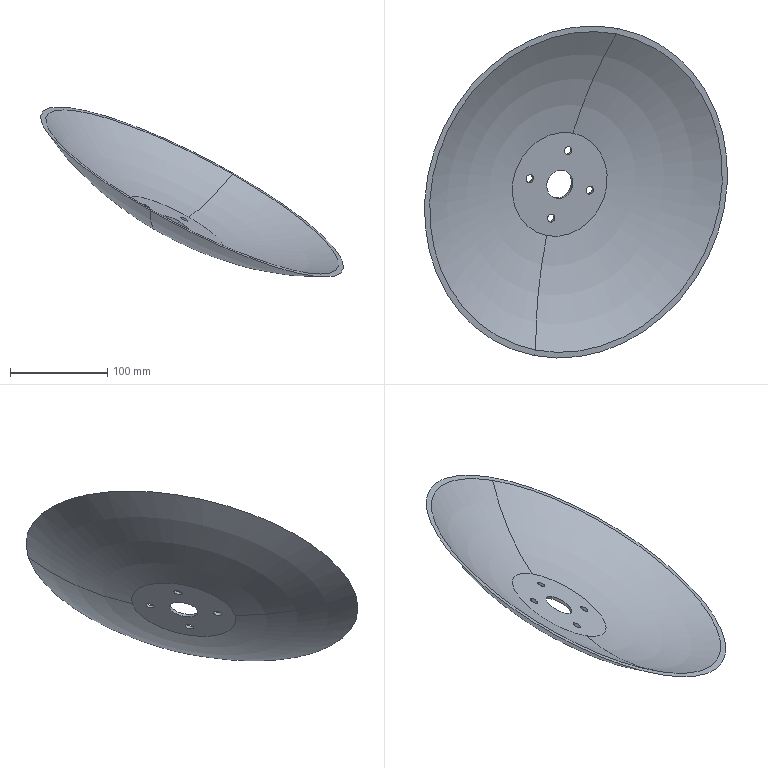Component | SolidWorks | AttachedSoilDiskDiameter350-2 | 1 solid | 17 faces | volume 294370 mm3 | cylinder 10 | torus 4 | plane 3 | commonest cylinder face diameters 8.5 x8 30 x2
STEP:
#1=COLOUR_RGB('',0.7922,0.8196,0.9333);
#2=FILL_AREA_STYLE_COLOUR('',#1);
#3=FILL_AREA_STYLE('',(#2));
#4=SURFACE_STYLE_FILL_AREA(#3);
#5=SURFACE_SIDE_STYLE('',(#4));
#6=SURFACE_STYLE_USAGE(.BOTH.,#5);
#7=PRESENTATION_STYLE_ASSIGNMENT((#6));
#8=CARTESIAN_POINT('',(-77.113,-11.399,41.303));
#9=VERTEX_POINT('',#8);
#10=CARTESIAN_POINT('',(-77.196,-11.721,41.266));
#11=VERTEX_POINT('',#10);
#12=CARTESIAN_POINT('',(-77.155,-11.56,41.285));
#13=DIRECTION('',(0.4522,-0.2133,0.866));
#14=DIRECTION('',(-0.2454,-0.9633,-0.1091));
#15=AXIS2_PLACEMENT_3D('',#12,#13,#14);
#16=CIRCLE('',#15,0.1673);
#17=EDGE_CURVE('',#9,#11,#16,.T.);
#18=ORIENTED_EDGE('',*,*,#17,.T.);
#19=CARTESIAN_POINT('',(-77.249,-11.696,41.164));
#20=VERTEX_POINT('',#19);
#21=CARTESIAN_POINT('',(-77.071,-11.78,41.505));
#22=DIRECTION('',(-0.4522,0.2133,-0.866));
#23=VECTOR('',#22,39.37);
#24=LINE('',#21,#23);
#25=EDGE_CURVE('',#11,#20,#24,.T.);
#26=ORIENTED_EDGE('',*,*,#25,.T.);
#27=CARTESIAN_POINT('',(-77.167,-11.374,41.201));
#28=VERTEX_POINT('',#27);
#29=CARTESIAN_POINT('',(-77.208,-11.535,41.182));
#30=DIRECTION('',(-0.4522,0.2133,-0.866));
#31=DIRECTION('',(-0.8575,0.1632,0.4879));
#32=AXIS2_PLACEMENT_3D('',#29,#30,#31);
#33=CIRCLE('',#32,0.1673);
#34=EDGE_CURVE('',#20,#28,#33,.T.);
#35=ORIENTED_EDGE('',*,*,#34,.T.);
#36=CARTESIAN_POINT('',(-76.989,-11.458,41.542));
#37=DIRECTION('',(-0.4522,0.2133,-0.866));
#38=VECTOR('',#37,39.37);
#39=LINE('',#36,#38);
#40=EDGE_CURVE('',#9,#28,#39,.T.);
#41=ORIENTED_EDGE('',*,*,#40,.F.);
#42=EDGE_LOOP('',(#18,#26,#35,#41));
#43=FACE_OUTER_BOUND('',#42,.T.);
#44=CARTESIAN_POINT('',(-77.03,-11.619,41.523));
#45=DIRECTION('',(-0.4522,0.2133,-0.866));
#46=DIRECTION('',(0.2454,0.9633,0.1091));
#47=AXIS2_PLACEMENT_3D('',#44,#45,#46);
#48=CYLINDRICAL_SURFACE('',#47,0.1673);
#49=ADVANCED_FACE('',(#43),#48,.F.);
#50=CARTESIAN_POINT('',(-76.246,-12.995,40.457));
#51=VERTEX_POINT('',#50);
#52=CARTESIAN_POINT('',(-76.328,-13.318,40.42));
#53=VERTEX_POINT('',#52);
#54=CARTESIAN_POINT('',(-76.287,-13.157,40.438));
#55=DIRECTION('',(0.4522,-0.2133,0.866));
#56=DIRECTION('',(-0.2454,-0.9633,-0.1091));
#57=AXIS2_PLACEMENT_3D('',#54,#55,#56);
#58=CIRCLE('',#57,0.1673);
#59=EDGE_CURVE('',#51,#53,#58,.T.);
#60=ORIENTED_EDGE('',*,*,#59,.T.);
#61=CARTESIAN_POINT('',(-76.381,-13.293,40.318));
#62=VERTEX_POINT('',#61);
#63=CARTESIAN_POINT('',(-76.203,-13.376,40.659));
#64=DIRECTION('',(-0.4522,0.2133,-0.866));
#65=VECTOR('',#64,39.37);
#66=LINE('',#63,#65);
#67=EDGE_CURVE('',#53,#62,#66,.T.);
#68=ORIENTED_EDGE('',*,*,#67,.T.);
#69=CARTESIAN_POINT('',(-76.299,-12.97,40.354));
#70=VERTEX_POINT('',#69);
#71=CARTESIAN_POINT('',(-76.34,-13.131,40.336));
#72=DIRECTION('',(-0.4522,0.2133,-0.866));
#73=DIRECTION('',(-0.2454,-0.9633,-0.1091));
#74=AXIS2_PLACEMENT_3D('',#71,#72,#73);
#75=CIRCLE('',#74,0.1673);
#76=EDGE_CURVE('',#62,#70,#75,.T.);
#77=ORIENTED_EDGE('',*,*,#76,.T.);
#78=CARTESIAN_POINT('',(-76.121,-13.054,40.695));
#79=DIRECTION('',(-0.4522,0.2133,-0.866));
#80=VECTOR('',#79,39.37);
#81=LINE('',#78,#80);
#82=EDGE_CURVE('',#51,#70,#81,.T.);
#83=ORIENTED_EDGE('',*,*,#82,.F.);
#84=EDGE_LOOP('',(#60,#68,#77,#83));
#85=FACE_OUTER_BOUND('',#84,.T.);
#86=CARTESIAN_POINT('',(-76.162,-13.215,40.677));
#87=DIRECTION('',(-0.4522,0.2133,-0.866));
#88=DIRECTION('',(0.2454,0.9633,0.1091));
#89=AXIS2_PLACEMENT_3D('',#86,#87,#88);
#90=CYLINDRICAL_SURFACE('',#89,0.1673);
#91=ADVANCED_FACE('',(#85),#90,.F.);
#92=CARTESIAN_POINT('',(-74.683,-11.861,39.92));
#93=VERTEX_POINT('',#92);
#94=CARTESIAN_POINT('',(-74.765,-12.184,39.883));
#95=VERTEX_POINT('',#94);
#96=CARTESIAN_POINT('',(-74.724,-12.023,39.901));
#97=DIRECTION('',(0.4522,-0.2133,0.866));
#98=DIRECTION('',(-0.2454,-0.9633,-0.1091));
#99=AXIS2_PLACEMENT_3D('',#96,#97,#98);
#100=CIRCLE('',#99,0.1673);
#101=EDGE_CURVE('',#93,#95,#100,.T.);
#102=ORIENTED_EDGE('',*,*,#101,.T.);
#103=CARTESIAN_POINT('',(-74.818,-12.159,39.781));
#104=VERTEX_POINT('',#103);
#105=CARTESIAN_POINT('',(-74.64,-12.242,40.122));
#106=DIRECTION('',(-0.4522,0.2133,-0.866));
#107=VECTOR('',#106,39.37);
#108=LINE('',#105,#107);
#109=EDGE_CURVE('',#95,#104,#108,.T.);
#110=ORIENTED_EDGE('',*,*,#109,.T.);
#111=CARTESIAN_POINT('',(-74.736,-11.836,39.817));
#112=VERTEX_POINT('',#111);
#113=CARTESIAN_POINT('',(-74.777,-11.997,39.799));
#114=DIRECTION('',(-0.4522,0.2133,-0.866));
#115=DIRECTION('',(0.8575,-0.1632,-0.4879));
#116=AXIS2_PLACEMENT_3D('',#113,#114,#115);
#117=CIRCLE('',#116,0.1673);
#118=EDGE_CURVE('',#104,#112,#117,.T.);
#119=ORIENTED_EDGE('',*,*,#118,.T.);
#120=CARTESIAN_POINT('',(-74.558,-11.92,40.158));
#121=DIRECTION('',(-0.4522,0.2133,-0.866));
#122=VECTOR('',#121,39.37);
#123=LINE('',#120,#122);
#124=EDGE_CURVE('',#93,#112,#123,.T.);
#125=ORIENTED_EDGE('',*,*,#124,.F.);
#126=EDGE_LOOP('',(#102,#110,#119,#125));
#127=FACE_OUTER_BOUND('',#126,.T.);
#128=CARTESIAN_POINT('',(-74.599,-12.081,40.14));
#129=DIRECTION('',(-0.4522,0.2133,-0.866));
#130=DIRECTION('',(0.2454,0.9633,0.1091));
#131=AXIS2_PLACEMENT_3D('',#128,#129,#130);
#132=CYLINDRICAL_SURFACE('',#131,0.1673);
#133=ADVANCED_FACE('',(#127),#132,.F.);
#134=CARTESIAN_POINT('',(-75.55,-10.265,40.766));
#135=VERTEX_POINT('',#134);
#136=CARTESIAN_POINT('',(-75.632,-10.587,40.729));
#137=VERTEX_POINT('',#136);
#138=CARTESIAN_POINT('',(-75.591,-10.426,40.748));
#139=DIRECTION('',(0.4522,-0.2133,0.866));
#140=DIRECTION('',(-0.2454,-0.9633,-0.1091));
#141=AXIS2_PLACEMENT_3D('',#138,#139,#140);
#142=CIRCLE('',#141,0.1673);
#143=EDGE_CURVE('',#135,#137,#142,.T.);
#144=ORIENTED_EDGE('',*,*,#143,.T.);
#145=CARTESIAN_POINT('',(-75.686,-10.562,40.627));
#146=VERTEX_POINT('',#145);
#147=CARTESIAN_POINT('',(-75.508,-10.646,40.968));
#148=DIRECTION('',(-0.4522,0.2133,-0.866));
#149=VECTOR('',#148,39.37);
#150=LINE('',#147,#149);
#151=EDGE_CURVE('',#137,#146,#150,.T.);
#152=ORIENTED_EDGE('',*,*,#151,.T.);
#153=CARTESIAN_POINT('',(-75.604,-10.24,40.664));
#154=VERTEX_POINT('',#153);
#155=CARTESIAN_POINT('',(-75.645,-10.401,40.645));
#156=DIRECTION('',(-0.4522,0.2133,-0.866));
#157=DIRECTION('',(0.2454,0.9633,0.1091));
#158=AXIS2_PLACEMENT_3D('',#155,#156,#157);
#159=CIRCLE('',#158,0.1673);
#160=EDGE_CURVE('',#146,#154,#159,.T.);
#161=ORIENTED_EDGE('',*,*,#160,.T.);
#162=CARTESIAN_POINT('',(-75.426,-10.324,41.005));
#163=DIRECTION('',(-0.4522,0.2133,-0.866));
#164=VECTOR('',#163,39.37);
#165=LINE('',#162,#164);
#166=EDGE_CURVE('',#135,#154,#165,.T.);
#167=ORIENTED_EDGE('',*,*,#166,.F.);
#168=EDGE_LOOP('',(#144,#152,#161,#167));
#169=FACE_OUTER_BOUND('',#168,.T.);
#170=CARTESIAN_POINT('',(-75.467,-10.485,40.986));
#171=DIRECTION('',(-0.4522,0.2133,-0.866));
#172=DIRECTION('',(0.2454,0.9633,0.1091));
#173=AXIS2_PLACEMENT_3D('',#170,#171,#172);
#174=CYLINDRICAL_SURFACE('',#173,0.1673);
#175=ADVANCED_FACE('',(#169),#174,.F.);
#176=CARTESIAN_POINT('',(-75.794,-11.222,40.657));
#177=VERTEX_POINT('',#176);
#178=CARTESIAN_POINT('',(-76.084,-12.36,40.529));
#179=VERTEX_POINT('',#178);
#180=CARTESIAN_POINT('',(-75.939,-11.791,40.593));
#181=DIRECTION('',(0.4522,-0.2133,0.866));
#182=DIRECTION('',(-0.2454,-0.9633,-0.1091));
#183=AXIS2_PLACEMENT_3D('',#180,#181,#182);
#184=CIRCLE('',#183,0.5906);
#185=EDGE_CURVE('',#177,#179,#184,.T.);
#186=ORIENTED_EDGE('',*,*,#185,.T.);
#187=CARTESIAN_POINT('',(-76.138,-12.335,40.426));
#188=VERTEX_POINT('',#187);
#189=CARTESIAN_POINT('',(-75.959,-12.419,40.767));
#190=DIRECTION('',(-0.4522,0.2133,-0.866));
#191=VECTOR('',#190,39.37);
#192=LINE('',#189,#191);
#193=EDGE_CURVE('',#179,#188,#192,.T.);
#194=ORIENTED_EDGE('',*,*,#193,.T.);
#195=CARTESIAN_POINT('',(-75.848,-11.197,40.555));
#196=VERTEX_POINT('',#195);
#197=CARTESIAN_POINT('',(-75.993,-11.766,40.491));
#198=DIRECTION('',(-0.4522,0.2133,-0.866));
#199=DIRECTION('',(0.2454,0.9633,0.1091));
#200=AXIS2_PLACEMENT_3D('',#197,#198,#199);
#201=CIRCLE('',#200,0.5906);
#202=EDGE_CURVE('',#188,#196,#201,.T.);
#203=ORIENTED_EDGE('',*,*,#202,.T.);
#204=CARTESIAN_POINT('',(-75.67,-11.281,40.896));
#205=DIRECTION('',(-0.4522,0.2133,-0.866));
#206=VECTOR('',#205,39.37);
#207=LINE('',#204,#206);
#208=EDGE_CURVE('',#177,#196,#207,.T.);
#209=ORIENTED_EDGE('',*,*,#208,.F.);
#210=EDGE_LOOP('',(#186,#194,#203,#209));
#211=FACE_OUTER_BOUND('',#210,.T.);
#212=CARTESIAN_POINT('',(-75.815,-11.85,40.832));
#213=DIRECTION('',(-0.4522,0.2133,-0.866));
#214=DIRECTION('',(0.2454,0.9633,0.1091));
#215=AXIS2_PLACEMENT_3D('',#212,#213,#214);
#216=CYLINDRICAL_SURFACE('',#215,0.5906);
#217=ADVANCED_FACE('',(#211),#216,.F.);
#218=CARTESIAN_POINT('',(-76.913,-18.512,41.128));
#219=VERTEX_POINT('',#218);
#220=CARTESIAN_POINT('',(-73.648,-5.692,42.581));
#221=VERTEX_POINT('',#220);
#222=CARTESIAN_POINT('',(-75.28,-12.102,41.855));
#223=DIRECTION('',(-0.4522,0.2133,-0.866));
#224=DIRECTION('',(0.2454,0.9633,0.1091));
#225=AXIS2_PLACEMENT_3D('',#222,#223,#224);
#226=CIRCLE('',#225,6.654);
#227=EDGE_CURVE('',#219,#221,#226,.T.);
#228=ORIENTED_EDGE('',*,*,#227,.F.);
#229=CARTESIAN_POINT('',(-76.469,-13.871,40.357));
#230=VERTEX_POINT('',#229);
#231=CARTESIAN_POINT('',(-70.898,-15.115,50.563));
#232=DIRECTION('',(0.8575,-0.1632,-0.4879));
#233=DIRECTION('',(-0.4946,0.,-0.8691));
#234=AXIS2_PLACEMENT_3D('',#231,#232,#233);
#235=CIRCLE('',#234,11.693);
#236=EDGE_CURVE('',#219,#230,#235,.T.);
#237=ORIENTED_EDGE('',*,*,#236,.T.);
#238=CARTESIAN_POINT('',(-75.409,-9.712,40.829));
#239=VERTEX_POINT('',#238);
#240=CARTESIAN_POINT('',(-75.939,-11.791,40.593));
#241=DIRECTION('',(-0.4522,0.2133,-0.866));
#242=DIRECTION('',(0.2454,0.9633,0.1091));
#243=AXIS2_PLACEMENT_3D('',#240,#241,#242);
#244=CIRCLE('',#243,2.159);
#245=EDGE_CURVE('',#230,#239,#244,.T.);
#246=ORIENTED_EDGE('',*,*,#245,.T.);
#247=CARTESIAN_POINT('',(-70.468,-13.426,50.754));
#248=DIRECTION('',(-0.8575,0.1632,0.4879));
#249=DIRECTION('',(0.4946,0.,0.8691));
#250=AXIS2_PLACEMENT_3D('',#247,#248,#249);
#251=CIRCLE('',#250,11.693);
#252=EDGE_CURVE('',#221,#239,#251,.T.);
#253=ORIENTED_EDGE('',*,*,#252,.F.);
#254=EDGE_LOOP('',(#228,#237,#246,#253));
#255=FACE_OUTER_BOUND('',#254,.T.);
#256=CARTESIAN_POINT('',(-70.683,-14.27,50.658));
#257=DIRECTION('',(-0.4522,0.2133,-0.866));
#258=DIRECTION('',(0.2454,0.9633,0.1091));
#259=AXIS2_PLACEMENT_3D('',#256,#257,#258);
#260=TOROIDAL_SURFACE('',#259,0.8765,11.693);
#261=ADVANCED_FACE('',(#255),#260,.F.);
#262=CARTESIAN_POINT('',(-73.59,-5.465,42.606));
#263=VERTEX_POINT('',#262);
#264=CARTESIAN_POINT('',(-76.971,-18.739,41.103));
#265=VERTEX_POINT('',#264);
#266=CARTESIAN_POINT('',(-75.28,-12.102,41.855));
#267=DIRECTION('',(-0.4522,0.2133,-0.866));
#268=DIRECTION('',(0.2454,0.9633,0.1091));
#269=AXIS2_PLACEMENT_3D('',#266,#267,#268);
#270=CIRCLE('',#269,6.89);
#271=EDGE_CURVE('',#263,#265,#270,.T.);
#272=ORIENTED_EDGE('',*,*,#271,.T.);
#273=CARTESIAN_POINT('',(-76.524,-13.852,40.254));
#274=VERTEX_POINT('',#273);
#275=CARTESIAN_POINT('',(-70.898,-15.115,50.563));
#276=DIRECTION('',(0.8575,-0.1632,-0.4879));
#277=DIRECTION('',(-0.4946,0.,-0.8691));
#278=AXIS2_PLACEMENT_3D('',#275,#276,#277);
#279=CIRCLE('',#278,11.811);
#280=EDGE_CURVE('',#265,#274,#279,.T.);
#281=ORIENTED_EDGE('',*,*,#280,.T.);
#282=CARTESIAN_POINT('',(-75.461,-9.68,40.727));
#283=VERTEX_POINT('',#282);
#284=CARTESIAN_POINT('',(-75.993,-11.766,40.491));
#285=DIRECTION('',(-0.4522,0.2133,-0.866));
#286=DIRECTION('',(0.2454,0.9633,0.1091));
#287=AXIS2_PLACEMENT_3D('',#284,#285,#286);
#288=CIRCLE('',#287,2.165);
#289=EDGE_CURVE('',#283,#274,#288,.T.);
#290=ORIENTED_EDGE('',*,*,#289,.F.);
#291=CARTESIAN_POINT('',(-70.468,-13.426,50.754));
#292=DIRECTION('',(-0.8575,0.1632,0.4879));
#293=DIRECTION('',(0.4946,0.,0.8691));
#294=AXIS2_PLACEMENT_3D('',#291,#292,#293);
#295=CIRCLE('',#294,11.811);
#296=EDGE_CURVE('',#263,#283,#295,.T.);
#297=ORIENTED_EDGE('',*,*,#296,.F.);
#298=EDGE_LOOP('',(#272,#281,#290,#297));
#299=FACE_OUTER_BOUND('',#298,.T.);
#300=CARTESIAN_POINT('',(-70.683,-14.27,50.658));
#301=DIRECTION('',(-0.4522,0.2133,-0.866));
#302=DIRECTION('',(0.2454,0.9633,0.1091));
#303=AXIS2_PLACEMENT_3D('',#300,#301,#302);
#304=TOROIDAL_SURFACE('',#303,0.8765,11.811);
#305=ADVANCED_FACE('',(#299),#304,.T.);
#306=ORIENTED_EDGE('',*,*,#280,.F.);
#307=CARTESIAN_POINT('',(-75.28,-12.102,41.855));
#308=DIRECTION('',(-0.4522,0.2133,-0.866));
#309=DIRECTION('',(0.2454,0.9633,0.1091));
#310=AXIS2_PLACEMENT_3D('',#307,#308,#309);
#311=CIRCLE('',#310,6.89);
#312=EDGE_CURVE('',#265,#263,#311,.T.);
#313=ORIENTED_EDGE('',*,*,#312,.T.);
#314=ORIENTED_EDGE('',*,*,#296,.T.);
#315=CARTESIAN_POINT('',(-75.993,-11.766,40.491));
#316=DIRECTION('',(-0.4522,0.2133,-0.866));
#317=DIRECTION('',(0.2454,0.9633,0.1091));
#318=AXIS2_PLACEMENT_3D('',#315,#316,#317);
#319=CIRCLE('',#318,2.165);
#320=EDGE_CURVE('',#274,#283,#319,.T.);
#321=ORIENTED_EDGE('',*,*,#320,.F.);
#322=EDGE_LOOP('',(#306,#313,#314,#321));
#323=FACE_OUTER_BOUND('',#322,.T.);
#324=CARTESIAN_POINT('',(-70.683,-14.27,50.658));
#325=DIRECTION('',(-0.4522,0.2133,-0.866));
#326=DIRECTION('',(0.2454,0.9633,0.1091));
#327=AXIS2_PLACEMENT_3D('',#324,#325,#326);
#328=TOROIDAL_SURFACE('',#327,0.8765,11.811);
#329=ADVANCED_FACE('',(#323),#328,.T.);
#330=CARTESIAN_POINT('',(-77.208,-11.535,41.182));
#331=DIRECTION('',(-0.4522,0.2133,-0.866));
#332=DIRECTION('',(-0.8575,0.1632,0.4879));
#333=AXIS2_PLACEMENT_3D('',#330,#331,#332);
#334=CIRCLE('',#333,0.1673);
#335=EDGE_CURVE('',#28,#20,#334,.T.);
#336=ORIENTED_EDGE('',*,*,#335,.F.);
#337=ORIENTED_EDGE('',*,*,#34,.F.);
#338=EDGE_LOOP('',(#336,#337));
#339=FACE_BOUND('',#338,.T.);
#340=CARTESIAN_POINT('',(-76.34,-13.131,40.336));
#341=DIRECTION('',(-0.4522,0.2133,-0.866));
#342=DIRECTION('',(-0.2454,-0.9633,-0.1091));
#343=AXIS2_PLACEMENT_3D('',#340,#341,#342);
#344=CIRCLE('',#343,0.1673);
#345=EDGE_CURVE('',#70,#62,#344,.T.);
#346=ORIENTED_EDGE('',*,*,#345,.F.);
#347=ORIENTED_EDGE('',*,*,#76,.F.);
#348=EDGE_LOOP('',(#346,#347));
#349=FACE_BOUND('',#348,.T.);
#350=CARTESIAN_POINT('',(-74.777,-11.997,39.799));
#351=DIRECTION('',(-0.4522,0.2133,-0.866));
#352=DIRECTION('',(0.8575,-0.1632,-0.4879));
#353=AXIS2_PLACEMENT_3D('',#350,#351,#352);
#354=CIRCLE('',#353,0.1673);
#355=EDGE_CURVE('',#112,#104,#354,.T.);
#356=ORIENTED_EDGE('',*,*,#355,.F.);
#357=ORIENTED_EDGE('',*,*,#118,.F.);
#358=EDGE_LOOP('',(#356,#357));
#359=FACE_BOUND('',#358,.T.);
#360=CARTESIAN_POINT('',(-75.645,-10.401,40.645));
#361=DIRECTION('',(-0.4522,0.2133,-0.866));
#362=DIRECTION('',(0.2454,0.9633,0.1091));
#363=AXIS2_PLACEMENT_3D('',#360,#361,#362);
#364=CIRCLE('',#363,0.1673);
#365=EDGE_CURVE('',#154,#146,#364,.T.);
#366=ORIENTED_EDGE('',*,*,#365,.F.);
#367=ORIENTED_EDGE('',*,*,#160,.F.);
#368=EDGE_LOOP('',(#366,#367));
#369=FACE_BOUND('',#368,.T.);
#370=CARTESIAN_POINT('',(-75.993,-11.766,40.491));
#371=DIRECTION('',(-0.4522,0.2133,-0.866));
#372=DIRECTION('',(0.2454,0.9633,0.1091));
#373=AXIS2_PLACEMENT_3D('',#370,#371,#372);
#374=CIRCLE('',#373,0.5906);
#375=EDGE_CURVE('',#196,#188,#374,.T.);
#376=ORIENTED_EDGE('',*,*,#375,.F.);
#377=ORIENTED_EDGE('',*,*,#202,.F.);
#378=EDGE_LOOP('',(#376,#377));
#379=FACE_BOUND('',#378,.T.);
#380=ORIENTED_EDGE('',*,*,#289,.T.);
#381=ORIENTED_EDGE('',*,*,#320,.T.);
#382=EDGE_LOOP('',(#380,#381));
#383=FACE_OUTER_BOUND('',#382,.T.);
#384=CARTESIAN_POINT('',(-75.461,-9.68,40.727));
#385=DIRECTION('',(-0.4522,0.2133,-0.866));
#386=DIRECTION('',(0.2454,0.9633,0.1091));
#387=AXIS2_PLACEMENT_3D('',#384,#385,#386);
#388=PLANE('',#387);
#389=ADVANCED_FACE('',(#339,#349,#359,#369,#379,#383),#388,.T.);
#390=ORIENTED_EDGE('',*,*,#17,.F.);
#391=CARTESIAN_POINT('',(-77.155,-11.56,41.285));
#392=DIRECTION('',(0.4522,-0.2133,0.866));
#393=DIRECTION('',(-0.2454,-0.9633,-0.1091));
#394=AXIS2_PLACEMENT_3D('',#391,#392,#393);
#395=CIRCLE('',#394,0.1673);
#396=EDGE_CURVE('',#11,#9,#395,.T.);
#397=ORIENTED_EDGE('',*,*,#396,.F.);
#398=EDGE_LOOP('',(#390,#397));
#399=FACE_BOUND('',#398,.T.);
#400=ORIENTED_EDGE('',*,*,#59,.F.);
#401=CARTESIAN_POINT('',(-76.287,-13.157,40.438));
#402=DIRECTION('',(0.4522,-0.2133,0.866));
#403=DIRECTION('',(-0.2454,-0.9633,-0.1091));
#404=AXIS2_PLACEMENT_3D('',#401,#402,#403);
#405=CIRCLE('',#404,0.1673);
#406=EDGE_CURVE('',#53,#51,#405,.T.);
#407=ORIENTED_EDGE('',*,*,#406,.F.);
#408=EDGE_LOOP('',(#400,#407));
#409=FACE_BOUND('',#408,.T.);
#410=ORIENTED_EDGE('',*,*,#101,.F.);
#411=CARTESIAN_POINT('',(-74.724,-12.023,39.901));
#412=DIRECTION('',(0.4522,-0.2133,0.866));
#413=DIRECTION('',(-0.2454,-0.9633,-0.1091));
#414=AXIS2_PLACEMENT_3D('',#411,#412,#413);
#415=CIRCLE('',#414,0.1673);
#416=EDGE_CURVE('',#95,#93,#415,.T.);
#417=ORIENTED_EDGE('',*,*,#416,.F.);
#418=EDGE_LOOP('',(#410,#417));
#419=FACE_BOUND('',#418,.T.);
#420=ORIENTED_EDGE('',*,*,#143,.F.);
#421=CARTESIAN_POINT('',(-75.591,-10.426,40.748));
#422=DIRECTION('',(0.4522,-0.2133,0.866));
#423=DIRECTION('',(-0.2454,-0.9633,-0.1091));
#424=AXIS2_PLACEMENT_3D('',#421,#422,#423);
#425=CIRCLE('',#424,0.1673);
#426=EDGE_CURVE('',#137,#135,#425,.T.);
#427=ORIENTED_EDGE('',*,*,#426,.F.);
#428=EDGE_LOOP('',(#420,#427));
#429=FACE_BOUND('',#428,.T.);
#430=ORIENTED_EDGE('',*,*,#185,.F.);
#431=CARTESIAN_POINT('',(-75.939,-11.791,40.593));
#432=DIRECTION('',(0.4522,-0.2133,0.866));
#433=DIRECTION('',(-0.2454,-0.9633,-0.1091));
#434=AXIS2_PLACEMENT_3D('',#431,#432,#433);
#435=CIRCLE('',#434,0.5906);
#436=EDGE_CURVE('',#179,#177,#435,.T.);
#437=ORIENTED_EDGE('',*,*,#436,.F.);
#438=EDGE_LOOP('',(#430,#437));
#439=FACE_BOUND('',#438,.T.);
#440=CARTESIAN_POINT('',(-75.939,-11.791,40.593));
#441=DIRECTION('',(-0.4522,0.2133,-0.866));
#442=DIRECTION('',(0.2454,0.9633,0.1091));
#443=AXIS2_PLACEMENT_3D('',#440,#441,#442);
#444=CIRCLE('',#443,2.159);
#445=EDGE_CURVE('',#239,#230,#444,.T.);
#446=ORIENTED_EDGE('',*,*,#445,.F.);
#447=ORIENTED_EDGE('',*,*,#245,.F.);
#448=EDGE_LOOP('',(#446,#447));
#449=FACE_OUTER_BOUND('',#448,.T.);
#450=CARTESIAN_POINT('',(-75.409,-9.712,40.829));
#451=DIRECTION('',(0.4522,-0.2133,0.866));
#452=DIRECTION('',(-0.2454,-0.9633,-0.1091));
#453=AXIS2_PLACEMENT_3D('',#450,#451,#452);
#454=PLANE('',#453);
#455=ADVANCED_FACE('',(#399,#409,#419,#429,#439,#449),#454,.T.);
#456=ORIENTED_EDGE('',*,*,#236,.F.);
#457=CARTESIAN_POINT('',(-75.28,-12.102,41.855));
#458=DIRECTION('',(-0.4522,0.2133,-0.866));
#459=DIRECTION('',(0.2454,0.9633,0.1091));
#460=AXIS2_PLACEMENT_3D('',#457,#458,#459);
#461=CIRCLE('',#460,6.654);
#462=EDGE_CURVE('',#221,#219,#461,.T.);
#463=ORIENTED_EDGE('',*,*,#462,.F.);
#464=ORIENTED_EDGE('',*,*,#252,.T.);
#465=ORIENTED_EDGE('',*,*,#445,.T.);
#466=EDGE_LOOP('',(#456,#463,#464,#465));
#467=FACE_OUTER_BOUND('',#466,.T.);
#468=CARTESIAN_POINT('',(-70.683,-14.27,50.658));
#469=DIRECTION('',(-0.4522,0.2133,-0.866));
#470=DIRECTION('',(0.2454,0.9633,0.1091));
#471=AXIS2_PLACEMENT_3D('',#468,#469,#470);
#472=TOROIDAL_SURFACE('',#471,0.8765,11.693);
#473=ADVANCED_FACE('',(#467),#472,.F.);
#474=ORIENTED_EDGE('',*,*,#462,.T.);
#475=ORIENTED_EDGE('',*,*,#227,.T.);
#476=EDGE_LOOP('',(#474,#475));
#477=FACE_BOUND('',#476,.T.);
#478=ORIENTED_EDGE('',*,*,#271,.F.);
#479=ORIENTED_EDGE('',*,*,#312,.F.);
#480=EDGE_LOOP('',(#478,#479));
#481=FACE_OUTER_BOUND('',#480,.T.);
#482=CARTESIAN_POINT('',(-73.648,-5.692,42.581));
#483=DIRECTION('',(0.4522,-0.2133,0.866));
#484=DIRECTION('',(-0.2454,-0.9633,-0.1091));
#485=AXIS2_PLACEMENT_3D('',#482,#483,#484);
#486=PLANE('',#485);
#487=ADVANCED_FACE('',(#477,#481),#486,.T.);
#488=ORIENTED_EDGE('',*,*,#193,.F.);
#489=ORIENTED_EDGE('',*,*,#436,.T.);
#490=ORIENTED_EDGE('',*,*,#208,.T.);
#491=ORIENTED_EDGE('',*,*,#375,.T.);
#492=EDGE_LOOP('',(#488,#489,#490,#491));
#493=FACE_OUTER_BOUND('',#492,.T.);
#494=CARTESIAN_POINT('',(-75.815,-11.85,40.832));
#495=DIRECTION('',(-0.4522,0.2133,-0.866));
#496=DIRECTION('',(0.2454,0.9633,0.1091));
#497=AXIS2_PLACEMENT_3D('',#494,#495,#496);
#498=CYLINDRICAL_SURFACE('',#497,0.5906);
#499=ADVANCED_FACE('',(#493),#498,.F.);
#500=ORIENTED_EDGE('',*,*,#151,.F.);
#501=ORIENTED_EDGE('',*,*,#426,.T.);
#502=ORIENTED_EDGE('',*,*,#166,.T.);
#503=ORIENTED_EDGE('',*,*,#365,.T.);
#504=EDGE_LOOP('',(#500,#501,#502,#503));
#505=FACE_OUTER_BOUND('',#504,.T.);
#506=CARTESIAN_POINT('',(-75.467,-10.485,40.986));
#507=DIRECTION('',(-0.4522,0.2133,-0.866));
#508=DIRECTION('',(0.2454,0.9633,0.1091));
#509=AXIS2_PLACEMENT_3D('',#506,#507,#508);
#510=CYLINDRICAL_SURFACE('',#509,0.1673);
#511=ADVANCED_FACE('',(#505),#510,.F.);
#512=ORIENTED_EDGE('',*,*,#109,.F.);
#513=ORIENTED_EDGE('',*,*,#416,.T.);
#514=ORIENTED_EDGE('',*,*,#124,.T.);
#515=ORIENTED_EDGE('',*,*,#355,.T.);
#516=EDGE_LOOP('',(#512,#513,#514,#515));
#517=FACE_OUTER_BOUND('',#516,.T.);
#518=CARTESIAN_POINT('',(-74.599,-12.081,40.14));
#519=DIRECTION('',(-0.4522,0.2133,-0.866));
#520=DIRECTION('',(0.2454,0.9633,0.1091));
#521=AXIS2_PLACEMENT_3D('',#518,#519,#520);
#522=CYLINDRICAL_SURFACE('',#521,0.1673);
#523=ADVANCED_FACE('',(#517),#522,.F.);
#524=ORIENTED_EDGE('',*,*,#67,.F.);
#525=ORIENTED_EDGE('',*,*,#406,.T.);
#526=ORIENTED_EDGE('',*,*,#82,.T.);
#527=ORIENTED_EDGE('',*,*,#345,.T.);
#528=EDGE_LOOP('',(#524,#525,#526,#527));
#529=FACE_OUTER_BOUND('',#528,.T.);
#530=CARTESIAN_POINT('',(-76.162,-13.215,40.677));
#531=DIRECTION('',(-0.4522,0.2133,-0.866));
#532=DIRECTION('',(0.2454,0.9633,0.1091));
#533=AXIS2_PLACEMENT_3D('',#530,#531,#532);
#534=CYLINDRICAL_SURFACE('',#533,0.1673);
#535=ADVANCED_FACE('',(#529),#534,.F.);
#536=ORIENTED_EDGE('',*,*,#25,.F.);
#537=ORIENTED_EDGE('',*,*,#396,.T.);
#538=ORIENTED_EDGE('',*,*,#40,.T.);
#539=ORIENTED_EDGE('',*,*,#335,.T.);
#540=EDGE_LOOP('',(#536,#537,#538,#539));
#541=FACE_OUTER_BOUND('',#540,.T.);
#542=CARTESIAN_POINT('',(-77.03,-11.619,41.523));
#543=DIRECTION('',(-0.4522,0.2133,-0.866));
#544=DIRECTION('',(0.2454,0.9633,0.1091));
#545=AXIS2_PLACEMENT_3D('',#542,#543,#544);
#546=CYLINDRICAL_SURFACE('',#545,0.1673);
#547=ADVANCED_FACE('',(#541),#546,.F.);
#548=CLOSED_SHELL('',(#49,#91,#133,#175,#217,#261,#305,#329,#389,#455,#473,#487,#499,#511,#523,#535,#547));
#549=MANIFOLD_SOLID_BREP('',#548);
#550=STYLED_ITEM('',(#7),#549);
#551=PRESENTATION_LAYER_ASSIGNMENT('','',(#550));
#552=(LENGTH_UNIT()NAMED_UNIT(*)SI_UNIT($,.METRE.));
#553=LENGTH_MEASURE_WITH_UNIT(LENGTH_MEASURE(0.0254),#552);
#554=DIMENSIONAL_EXPONENTS(1.,0.,0.,0.,0.,0.,0.);
#555=(CONVERSION_BASED_UNIT('',#553)LENGTH_UNIT()NAMED_UNIT(#554));
#556=UNCERTAINTY_MEASURE_WITH_UNIT(LENGTH_MEASURE(0.00001),#555,'','');
#557=(NAMED_UNIT(*)PLANE_ANGLE_UNIT()SI_UNIT($,.RADIAN.));
#558=(NAMED_UNIT(*)SI_UNIT($,.STERADIAN.)SOLID_ANGLE_UNIT());
#559=(GEOMETRIC_REPRESENTATION_CONTEXT(3)GLOBAL_UNCERTAINTY_ASSIGNED_CONTEXT((#556))GLOBAL_UNIT_ASSIGNED_CONTEXT((#555,#557,#558))REPRESENTATION_CONTEXT('',''));
#560=MECHANICAL_DESIGN_GEOMETRIC_PRESENTATION_REPRESENTATION('',(#550),#559);
#561=CARTESIAN_POINT('',(0.,0.,0.));
#562=DIRECTION('',(0.,0.,1.));
#563=DIRECTION('',(1.,0.,0.));
#564=AXIS2_PLACEMENT_3D('',#561,#562,#563);
#565=(LENGTH_UNIT()NAMED_UNIT(*)SI_UNIT($,.METRE.));
#566=LENGTH_MEASURE_WITH_UNIT(LENGTH_MEASURE(0.0254),#565);
#567=DIMENSIONAL_EXPONENTS(1.,0.,0.,0.,0.,0.,0.);
#568=(CONVERSION_BASED_UNIT('',#566)LENGTH_UNIT()NAMED_UNIT(#567));
#569=UNCERTAINTY_MEASURE_WITH_UNIT(LENGTH_MEASURE(0.00001),#568,'','');
#570=(NAMED_UNIT(*)PLANE_ANGLE_UNIT()SI_UNIT($,.RADIAN.));
#571=(NAMED_UNIT(*)SI_UNIT($,.STERADIAN.)SOLID_ANGLE_UNIT());
#572=(GEOMETRIC_REPRESENTATION_CONTEXT(3)GLOBAL_UNCERTAINTY_ASSIGNED_CONTEXT((#569))GLOBAL_UNIT_ASSIGNED_CONTEXT((#568,#570,#571))REPRESENTATION_CONTEXT('',''));
#573=ADVANCED_BREP_SHAPE_REPRESENTATION('',(#549,#564),#572);